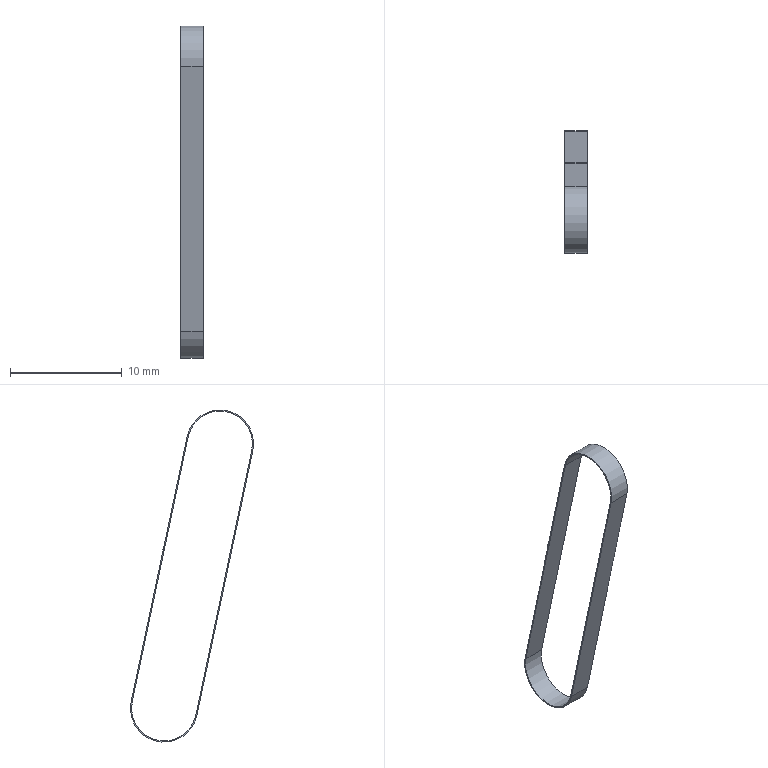Component | NX | BELT | 2 solids | 16 faces | box 2 x 11 x 29.68 mm | volume 13 mm3 | plane 12 | cylinder 4 | commonest cylinder face diameters 6 x2 5.8 x2
STEP:
#1=CARTESIAN_POINT('',(0.,0.,0.));
#2=DIRECTION('',(0.,0.,1.));
#3=DIRECTION('',(1.,0.,0.));
#4=AXIS2_PLACEMENT_3D('',#1,#2,#3);
#5=CARTESIAN_POINT('',(-47.1,-0.6394,30.62));
#6=VERTEX_POINT('',#5);
#7=CARTESIAN_POINT('',(-47.1,4.361,6.942));
#8=VERTEX_POINT('',#7);
#9=CARTESIAN_POINT('',(-47.1,4.361,6.942));
#10=DIRECTION('',(0.,0.2066,-0.9784));
#11=VECTOR('',#10,1.);
#12=LINE('',#9,#11);
#13=CARTESIAN_POINT('',(-47.1,4.263,6.921));
#14=DIRECTION('',(1.,0.,0.));
#15=DIRECTION('',(0.,-0.2066,0.9784));
#16=AXIS2_PLACEMENT_3D('',#13,#14,#15);
#17=PLANE('',#16);
#18=CARTESIAN_POINT('',(-0.,-0.1));
#19=DIRECTION('',(-1.,0.));
#20=VECTOR('',#19,1.);
#21=LINE('',#18,#20);
#22=(GEOMETRIC_REPRESENTATION_CONTEXT(2)PARAMETRIC_REPRESENTATION_CONTEXT()REPRESENTATION_CONTEXT('',''));
#23=DEFINITIONAL_REPRESENTATION('',(#21),#22);
#24=PCURVE('',#17,#23);
#25=CARTESIAN_POINT('',(-45.1,4.361,6.942));
#26=DIRECTION('',(0.,-0.9784,-0.2066));
#27=DIRECTION('',(1.,0.,0.));
#28=AXIS2_PLACEMENT_3D('',#25,#26,#27);
#29=PLANE('',#28);
#30=CARTESIAN_POINT('',(-2.,0.));
#31=DIRECTION('',(0.,-1.));
#32=VECTOR('',#31,1.);
#33=LINE('',#30,#32);
#34=(GEOMETRIC_REPRESENTATION_CONTEXT(2)PARAMETRIC_REPRESENTATION_CONTEXT()REPRESENTATION_CONTEXT('',''));
#35=DEFINITIONAL_REPRESENTATION('',(#33),#34);
#36=PCURVE('',#29,#35);
#37=SURFACE_CURVE('',#12,(#24,#36),.PCURVE_S1.);
#38=EDGE_CURVE('',#6,#8,#37,.T.);
#39=ORIENTED_EDGE('',*,*,#38,.T.);
#40=CARTESIAN_POINT('',(-47.1,-1.51,5.702));
#41=VERTEX_POINT('',#40);
#42=CARTESIAN_POINT('',(-47.1,1.425,6.322));
#43=DIRECTION('',(-1.,0.,0.));
#44=DIRECTION('',(0.,-0.9784,-0.2066));
#45=AXIS2_PLACEMENT_3D('',#42,#43,#44);
#46=CIRCLE('',#45,3.);
#47=CARTESIAN_POINT('',(-0.,5.9));
#48=CARTESIAN_POINT('',(5.196,5.9));
#49=CARTESIAN_POINT('',(2.598,1.4));
#50=CARTESIAN_POINT('',(-0.,-3.1));
#51=CARTESIAN_POINT('',(-2.598,1.4));
#52=CARTESIAN_POINT('',(-5.196,5.9));
#53=CARTESIAN_POINT('',(-0.,5.9));
#54=(BOUNDED_CURVE()B_SPLINE_CURVE(2,(#47,#48,#49,#50,#51,#52,#53),.UNSPECIFIED.,.T.,.F.)B_SPLINE_CURVE_WITH_KNOTS((1,2,2,2,2,1),(-2.094,0.,2.094,4.189,6.283,8.378),.UNSPECIFIED.)CURVE()GEOMETRIC_REPRESENTATION_ITEM()RATIONAL_B_SPLINE_CURVE((1.,0.5,1.,0.5,1.,0.5,1.))REPRESENTATION_ITEM(''));
#55=(GEOMETRIC_REPRESENTATION_CONTEXT(2)PARAMETRIC_REPRESENTATION_CONTEXT()REPRESENTATION_CONTEXT('',''));
#56=DEFINITIONAL_REPRESENTATION('',(#54),#55);
#57=PCURVE('',#17,#56);
#58=CARTESIAN_POINT('',(-45.1,1.425,6.322));
#59=DIRECTION('',(-1.,0.,0.));
#60=DIRECTION('',(0.,-0.9784,-0.2066));
#61=AXIS2_PLACEMENT_3D('',#58,#59,#60);
#62=CYLINDRICAL_SURFACE('',#61,3.);
#63=CARTESIAN_POINT('',(0.,2.));
#64=DIRECTION('',(1.,0.));
#65=VECTOR('',#64,1.);
#66=LINE('',#63,#65);
#67=(GEOMETRIC_REPRESENTATION_CONTEXT(2)PARAMETRIC_REPRESENTATION_CONTEXT()REPRESENTATION_CONTEXT('',''));
#68=DEFINITIONAL_REPRESENTATION('',(#66),#67);
#69=PCURVE('',#62,#68);
#70=SURFACE_CURVE('',#46,(#57,#69),.PCURVE_S1.);
#71=EDGE_CURVE('',#8,#41,#70,.T.);
#72=ORIENTED_EDGE('',*,*,#71,.T.);
#73=CARTESIAN_POINT('',(-47.1,-6.51,29.38));
#74=VERTEX_POINT('',#73);
#75=CARTESIAN_POINT('',(-47.1,-6.51,29.38));
#76=DIRECTION('',(0.,-0.2066,0.9784));
#77=VECTOR('',#76,1.);
#78=LINE('',#75,#77);
#79=CARTESIAN_POINT('',(24.2,5.9));
#80=DIRECTION('',(1.,0.));
#81=VECTOR('',#80,1.);
#82=LINE('',#79,#81);
#83=(GEOMETRIC_REPRESENTATION_CONTEXT(2)PARAMETRIC_REPRESENTATION_CONTEXT()REPRESENTATION_CONTEXT('',''));
#84=DEFINITIONAL_REPRESENTATION('',(#82),#83);
#85=PCURVE('',#17,#84);
#86=CARTESIAN_POINT('',(-45.1,-6.51,29.38));
#87=DIRECTION('',(0.,0.9784,0.2066));
#88=DIRECTION('',(-1.,0.,0.));
#89=AXIS2_PLACEMENT_3D('',#86,#87,#88);
#90=PLANE('',#89);
#91=CARTESIAN_POINT('',(2.,0.));
#92=DIRECTION('',(0.,1.));
#93=VECTOR('',#92,1.);
#94=LINE('',#91,#93);
#95=(GEOMETRIC_REPRESENTATION_CONTEXT(2)PARAMETRIC_REPRESENTATION_CONTEXT()REPRESENTATION_CONTEXT('',''));
#96=DEFINITIONAL_REPRESENTATION('',(#94),#95);
#97=PCURVE('',#90,#96);
#98=SURFACE_CURVE('',#78,(#85,#97),.PCURVE_S1.);
#99=EDGE_CURVE('',#41,#74,#98,.T.);
#100=ORIENTED_EDGE('',*,*,#99,.T.);
#101=CARTESIAN_POINT('',(-47.1,-3.575,30.));
#102=DIRECTION('',(-1.,0.,0.));
#103=DIRECTION('',(0.,-0.9784,-0.2066));
#104=AXIS2_PLACEMENT_3D('',#101,#102,#103);
#105=CIRCLE('',#104,3.);
#106=CARTESIAN_POINT('',(24.2,5.9));
#107=CARTESIAN_POINT('',(29.396,5.9));
#108=CARTESIAN_POINT('',(26.798,1.4));
#109=CARTESIAN_POINT('',(24.2,-3.1));
#110=CARTESIAN_POINT('',(21.602,1.4));
#111=CARTESIAN_POINT('',(19.004,5.9));
#112=CARTESIAN_POINT('',(24.2,5.9));
#113=(BOUNDED_CURVE()B_SPLINE_CURVE(2,(#106,#107,#108,#109,#110,#111,#112),.UNSPECIFIED.,.T.,.F.)B_SPLINE_CURVE_WITH_KNOTS((1,2,2,2,2,1),(-2.094,0.,2.094,4.189,6.283,8.378),.UNSPECIFIED.)CURVE()GEOMETRIC_REPRESENTATION_ITEM()RATIONAL_B_SPLINE_CURVE((1.,0.5,1.,0.5,1.,0.5,1.))REPRESENTATION_ITEM(''));
#114=(GEOMETRIC_REPRESENTATION_CONTEXT(2)PARAMETRIC_REPRESENTATION_CONTEXT()REPRESENTATION_CONTEXT('',''));
#115=DEFINITIONAL_REPRESENTATION('',(#113),#114);
#116=PCURVE('',#17,#115);
#117=CARTESIAN_POINT('',(-45.1,-3.575,30.));
#118=DIRECTION('',(-1.,0.,0.));
#119=DIRECTION('',(0.,-0.9784,-0.2066));
#120=AXIS2_PLACEMENT_3D('',#117,#118,#119);
#121=CYLINDRICAL_SURFACE('',#120,3.);
#122=CARTESIAN_POINT('',(0.,2.));
#123=DIRECTION('',(1.,0.));
#124=VECTOR('',#123,1.);
#125=LINE('',#122,#124);
#126=(GEOMETRIC_REPRESENTATION_CONTEXT(2)PARAMETRIC_REPRESENTATION_CONTEXT()REPRESENTATION_CONTEXT('',''));
#127=DEFINITIONAL_REPRESENTATION('',(#125),#126);
#128=PCURVE('',#121,#127);
#129=SURFACE_CURVE('',#105,(#116,#128),.PCURVE_S1.);
#130=EDGE_CURVE('',#74,#6,#129,.T.);
#131=ORIENTED_EDGE('',*,*,#130,.T.);
#132=EDGE_LOOP('',(#39,#72,#100,#131));
#133=FACE_BOUND('',#132,.T.);
#134=CARTESIAN_POINT('',(-47.1,4.263,6.921));
#135=VERTEX_POINT('',#134);
#136=CARTESIAN_POINT('',(-47.1,-0.7372,30.599));
#137=VERTEX_POINT('',#136);
#138=CARTESIAN_POINT('',(-47.1,4.263,6.921));
#139=DIRECTION('',(0.,-0.2066,0.9784));
#140=VECTOR('',#139,1.);
#141=LINE('',#138,#140);
#142=CARTESIAN_POINT('',(0.,0.));
#143=DIRECTION('',(1.,0.));
#144=VECTOR('',#143,1.);
#145=LINE('',#142,#144);
#146=(GEOMETRIC_REPRESENTATION_CONTEXT(2)PARAMETRIC_REPRESENTATION_CONTEXT()REPRESENTATION_CONTEXT('',''));
#147=DEFINITIONAL_REPRESENTATION('',(#145),#146);
#148=PCURVE('',#17,#147);
#149=CARTESIAN_POINT('',(-45.1,4.263,6.921));
#150=DIRECTION('',(0.,-0.9784,-0.2066));
#151=DIRECTION('',(1.,0.,0.));
#152=AXIS2_PLACEMENT_3D('',#149,#150,#151);
#153=PLANE('',#152);
#154=CARTESIAN_POINT('',(-2.,0.));
#155=DIRECTION('',(0.,1.));
#156=VECTOR('',#155,1.);
#157=LINE('',#154,#156);
#158=(GEOMETRIC_REPRESENTATION_CONTEXT(2)PARAMETRIC_REPRESENTATION_CONTEXT()REPRESENTATION_CONTEXT('',''));
#159=DEFINITIONAL_REPRESENTATION('',(#157),#158);
#160=PCURVE('',#153,#159);
#161=SURFACE_CURVE('',#141,(#148,#160),.PCURVE_S1.);
#162=EDGE_CURVE('',#135,#137,#161,.T.);
#163=ORIENTED_EDGE('',*,*,#162,.T.);
#164=CARTESIAN_POINT('',(-47.1,-6.412,29.401));
#165=VERTEX_POINT('',#164);
#166=CARTESIAN_POINT('',(-47.1,-3.575,30.));
#167=DIRECTION('',(1.,0.,0.));
#168=DIRECTION('',(0.,0.2066,-0.9784));
#169=AXIS2_PLACEMENT_3D('',#166,#167,#168);
#170=CIRCLE('',#169,2.9);
#171=CARTESIAN_POINT('',(24.2,2.9));
#172=DIRECTION('',(-1.,0.));
#173=AXIS2_PLACEMENT_2D('',#171,#172);
#174=CIRCLE('',#173,2.9);
#175=(GEOMETRIC_REPRESENTATION_CONTEXT(2)PARAMETRIC_REPRESENTATION_CONTEXT()REPRESENTATION_CONTEXT('',''));
#176=DEFINITIONAL_REPRESENTATION('',(#174),#175);
#177=PCURVE('',#17,#176);
#178=CARTESIAN_POINT('',(-45.1,-3.575,30.));
#179=DIRECTION('',(-1.,0.,0.));
#180=DIRECTION('',(0.,-0.9784,-0.2066));
#181=AXIS2_PLACEMENT_3D('',#178,#179,#180);
#182=CYLINDRICAL_SURFACE('',#181,2.9);
#183=CARTESIAN_POINT('',(4.712,2.));
#184=DIRECTION('',(-1.,0.));
#185=VECTOR('',#184,1.);
#186=LINE('',#183,#185);
#187=(GEOMETRIC_REPRESENTATION_CONTEXT(2)PARAMETRIC_REPRESENTATION_CONTEXT()REPRESENTATION_CONTEXT('',''));
#188=DEFINITIONAL_REPRESENTATION('',(#186),#187);
#189=PCURVE('',#182,#188);
#190=SURFACE_CURVE('',#170,(#177,#189),.PCURVE_S1.);
#191=EDGE_CURVE('',#137,#165,#190,.T.);
#192=ORIENTED_EDGE('',*,*,#191,.T.);
#193=CARTESIAN_POINT('',(-47.1,-1.412,5.723));
#194=VERTEX_POINT('',#193);
#195=CARTESIAN_POINT('',(-47.1,-6.412,29.401));
#196=DIRECTION('',(0.,0.2066,-0.9784));
#197=VECTOR('',#196,1.);
#198=LINE('',#195,#197);
#199=CARTESIAN_POINT('',(24.2,5.8));
#200=DIRECTION('',(-1.,0.));
#201=VECTOR('',#200,1.);
#202=LINE('',#199,#201);
#203=(GEOMETRIC_REPRESENTATION_CONTEXT(2)PARAMETRIC_REPRESENTATION_CONTEXT()REPRESENTATION_CONTEXT('',''));
#204=DEFINITIONAL_REPRESENTATION('',(#202),#203);
#205=PCURVE('',#17,#204);
#206=CARTESIAN_POINT('',(-45.1,-6.412,29.401));
#207=DIRECTION('',(0.,0.9784,0.2066));
#208=DIRECTION('',(-1.,0.,0.));
#209=AXIS2_PLACEMENT_3D('',#206,#207,#208);
#210=PLANE('',#209);
#211=CARTESIAN_POINT('',(2.,0.));
#212=DIRECTION('',(0.,-1.));
#213=VECTOR('',#212,1.);
#214=LINE('',#211,#213);
#215=(GEOMETRIC_REPRESENTATION_CONTEXT(2)PARAMETRIC_REPRESENTATION_CONTEXT()REPRESENTATION_CONTEXT('',''));
#216=DEFINITIONAL_REPRESENTATION('',(#214),#215);
#217=PCURVE('',#210,#216);
#218=SURFACE_CURVE('',#198,(#205,#217),.PCURVE_S1.);
#219=EDGE_CURVE('',#165,#194,#218,.T.);
#220=ORIENTED_EDGE('',*,*,#219,.T.);
#221=CARTESIAN_POINT('',(-47.1,1.425,6.322));
#222=DIRECTION('',(1.,0.,0.));
#223=DIRECTION('',(0.,-0.2066,0.9784));
#224=AXIS2_PLACEMENT_3D('',#221,#222,#223);
#225=CIRCLE('',#224,2.9);
#226=CARTESIAN_POINT('',(-0.,2.9));
#227=DIRECTION('',(1.,0.));
#228=AXIS2_PLACEMENT_2D('',#226,#227);
#229=CIRCLE('',#228,2.9);
#230=(GEOMETRIC_REPRESENTATION_CONTEXT(2)PARAMETRIC_REPRESENTATION_CONTEXT()REPRESENTATION_CONTEXT('',''));
#231=DEFINITIONAL_REPRESENTATION('',(#229),#230);
#232=PCURVE('',#17,#231);
#233=CARTESIAN_POINT('',(-45.1,1.425,6.322));
#234=DIRECTION('',(-1.,0.,0.));
#235=DIRECTION('',(0.,-0.9784,-0.2066));
#236=AXIS2_PLACEMENT_3D('',#233,#234,#235);
#237=CYLINDRICAL_SURFACE('',#236,2.9);
#238=CARTESIAN_POINT('',(7.854,2.));
#239=DIRECTION('',(-1.,0.));
#240=VECTOR('',#239,1.);
#241=LINE('',#238,#240);
#242=(GEOMETRIC_REPRESENTATION_CONTEXT(2)PARAMETRIC_REPRESENTATION_CONTEXT()REPRESENTATION_CONTEXT('',''));
#243=DEFINITIONAL_REPRESENTATION('',(#241),#242);
#244=PCURVE('',#237,#243);
#245=SURFACE_CURVE('',#225,(#232,#244),.PCURVE_S1.);
#246=EDGE_CURVE('',#194,#135,#245,.T.);
#247=ORIENTED_EDGE('',*,*,#246,.T.);
#248=EDGE_LOOP('',(#163,#192,#220,#247));
#249=FACE_BOUND('',#248,.T.);
#250=ADVANCED_FACE('',(#133,#249),#17,.F.);
#251=CARTESIAN_POINT('',(-45.1,-1.51,5.702));
#252=VERTEX_POINT('',#251);
#253=CARTESIAN_POINT('',(-45.1,-6.51,29.38));
#254=VERTEX_POINT('',#253);
#255=CARTESIAN_POINT('',(-45.1,-6.51,29.38));
#256=DIRECTION('',(0.,-0.2066,0.9784));
#257=VECTOR('',#256,1.);
#258=LINE('',#255,#257);
#259=CARTESIAN_POINT('',(-45.1,-6.412,29.401));
#260=DIRECTION('',(1.,0.,0.));
#261=DIRECTION('',(0.,0.2066,-0.9784));
#262=AXIS2_PLACEMENT_3D('',#259,#260,#261);
#263=PLANE('',#262);
#264=CARTESIAN_POINT('',(0.,-0.1));
#265=DIRECTION('',(-1.,0.));
#266=VECTOR('',#265,1.);
#267=LINE('',#264,#266);
#268=(GEOMETRIC_REPRESENTATION_CONTEXT(2)PARAMETRIC_REPRESENTATION_CONTEXT()REPRESENTATION_CONTEXT('',''));
#269=DEFINITIONAL_REPRESENTATION('',(#267),#268);
#270=PCURVE('',#263,#269);
#271=CARTESIAN_POINT('',(0.,0.));
#272=DIRECTION('',(0.,1.));
#273=VECTOR('',#272,1.);
#274=LINE('',#271,#273);
#275=(GEOMETRIC_REPRESENTATION_CONTEXT(2)PARAMETRIC_REPRESENTATION_CONTEXT()REPRESENTATION_CONTEXT('',''));
#276=DEFINITIONAL_REPRESENTATION('',(#274),#275);
#277=PCURVE('',#90,#276);
#278=SURFACE_CURVE('',#258,(#270,#277),.PCURVE_S1.);
#279=EDGE_CURVE('',#252,#254,#278,.T.);
#280=ORIENTED_EDGE('',*,*,#279,.F.);
#281=CARTESIAN_POINT('',(-45.1,4.361,6.942));
#282=VERTEX_POINT('',#281);
#283=CARTESIAN_POINT('',(-45.1,1.425,6.322));
#284=DIRECTION('',(-1.,0.,0.));
#285=DIRECTION('',(0.,-0.9784,-0.2066));
#286=AXIS2_PLACEMENT_3D('',#283,#284,#285);
#287=CIRCLE('',#286,3.);
#288=CARTESIAN_POINT('',(24.2,-0.1));
#289=CARTESIAN_POINT('',(19.004,-0.1));
#290=CARTESIAN_POINT('',(21.602,4.4));
#291=CARTESIAN_POINT('',(24.2,8.9));
#292=CARTESIAN_POINT('',(26.798,4.4));
#293=CARTESIAN_POINT('',(29.396,-0.1));
#294=CARTESIAN_POINT('',(24.2,-0.1));
#295=(BOUNDED_CURVE()B_SPLINE_CURVE(2,(#288,#289,#290,#291,#292,#293,#294),.UNSPECIFIED.,.T.,.F.)B_SPLINE_CURVE_WITH_KNOTS((1,2,2,2,2,1),(-2.094,0.,2.094,4.189,6.283,8.378),.UNSPECIFIED.)CURVE()GEOMETRIC_REPRESENTATION_ITEM()RATIONAL_B_SPLINE_CURVE((1.,0.5,1.,0.5,1.,0.5,1.))REPRESENTATION_ITEM(''));
#296=(GEOMETRIC_REPRESENTATION_CONTEXT(2)PARAMETRIC_REPRESENTATION_CONTEXT()REPRESENTATION_CONTEXT('',''));
#297=DEFINITIONAL_REPRESENTATION('',(#295),#296);
#298=PCURVE('',#263,#297);
#299=CARTESIAN_POINT('',(0.,0.));
#300=DIRECTION('',(1.,0.));
#301=VECTOR('',#300,1.);
#302=LINE('',#299,#301);
#303=(GEOMETRIC_REPRESENTATION_CONTEXT(2)PARAMETRIC_REPRESENTATION_CONTEXT()REPRESENTATION_CONTEXT('',''));
#304=DEFINITIONAL_REPRESENTATION('',(#302),#303);
#305=PCURVE('',#62,#304);
#306=SURFACE_CURVE('',#287,(#298,#305),.PCURVE_S1.);
#307=EDGE_CURVE('',#282,#252,#306,.T.);
#308=ORIENTED_EDGE('',*,*,#307,.F.);
#309=CARTESIAN_POINT('',(-45.1,-0.6394,30.62));
#310=VERTEX_POINT('',#309);
#311=CARTESIAN_POINT('',(-45.1,4.361,6.942));
#312=DIRECTION('',(0.,0.2066,-0.9784));
#313=VECTOR('',#312,1.);
#314=LINE('',#311,#313);
#315=CARTESIAN_POINT('',(24.2,5.9));
#316=DIRECTION('',(1.,0.));
#317=VECTOR('',#316,1.);
#318=LINE('',#315,#317);
#319=(GEOMETRIC_REPRESENTATION_CONTEXT(2)PARAMETRIC_REPRESENTATION_CONTEXT()REPRESENTATION_CONTEXT('',''));
#320=DEFINITIONAL_REPRESENTATION('',(#318),#319);
#321=PCURVE('',#263,#320);
#322=CARTESIAN_POINT('',(0.,0.));
#323=DIRECTION('',(0.,-1.));
#324=VECTOR('',#323,1.);
#325=LINE('',#322,#324);
#326=(GEOMETRIC_REPRESENTATION_CONTEXT(2)PARAMETRIC_REPRESENTATION_CONTEXT()REPRESENTATION_CONTEXT('',''));
#327=DEFINITIONAL_REPRESENTATION('',(#325),#326);
#328=PCURVE('',#29,#327);
#329=SURFACE_CURVE('',#314,(#321,#328),.PCURVE_S1.);
#330=EDGE_CURVE('',#310,#282,#329,.T.);
#331=ORIENTED_EDGE('',*,*,#330,.F.);
#332=CARTESIAN_POINT('',(-45.1,-3.575,30.));
#333=DIRECTION('',(-1.,0.,0.));
#334=DIRECTION('',(0.,-0.9784,-0.2066));
#335=AXIS2_PLACEMENT_3D('',#332,#333,#334);
#336=CIRCLE('',#335,3.);
#337=CARTESIAN_POINT('',(0.,-0.1));
#338=CARTESIAN_POINT('',(-5.196,-0.1));
#339=CARTESIAN_POINT('',(-2.598,4.4));
#340=CARTESIAN_POINT('',(0.,8.9));
#341=CARTESIAN_POINT('',(2.598,4.4));
#342=CARTESIAN_POINT('',(5.196,-0.1));
#343=CARTESIAN_POINT('',(0.,-0.1));
#344=(BOUNDED_CURVE()B_SPLINE_CURVE(2,(#337,#338,#339,#340,#341,#342,#343),.UNSPECIFIED.,.T.,.F.)B_SPLINE_CURVE_WITH_KNOTS((1,2,2,2,2,1),(-2.094,0.,2.094,4.189,6.283,8.378),.UNSPECIFIED.)CURVE()GEOMETRIC_REPRESENTATION_ITEM()RATIONAL_B_SPLINE_CURVE((1.,0.5,1.,0.5,1.,0.5,1.))REPRESENTATION_ITEM(''));
#345=(GEOMETRIC_REPRESENTATION_CONTEXT(2)PARAMETRIC_REPRESENTATION_CONTEXT()REPRESENTATION_CONTEXT('',''));
#346=DEFINITIONAL_REPRESENTATION('',(#344),#345);
#347=PCURVE('',#263,#346);
#348=CARTESIAN_POINT('',(0.,0.));
#349=DIRECTION('',(1.,0.));
#350=VECTOR('',#349,1.);
#351=LINE('',#348,#350);
#352=(GEOMETRIC_REPRESENTATION_CONTEXT(2)PARAMETRIC_REPRESENTATION_CONTEXT()REPRESENTATION_CONTEXT('',''));
#353=DEFINITIONAL_REPRESENTATION('',(#351),#352);
#354=PCURVE('',#121,#353);
#355=SURFACE_CURVE('',#336,(#347,#354),.PCURVE_S1.);
#356=EDGE_CURVE('',#254,#310,#355,.T.);
#357=ORIENTED_EDGE('',*,*,#356,.F.);
#358=EDGE_LOOP('',(#280,#308,#331,#357));
#359=FACE_BOUND('',#358,.T.);
#360=CARTESIAN_POINT('',(-45.1,-6.412,29.401));
#361=VERTEX_POINT('',#360);
#362=CARTESIAN_POINT('',(-45.1,-1.412,5.723));
#363=VERTEX_POINT('',#362);
#364=CARTESIAN_POINT('',(-45.1,-6.412,29.401));
#365=DIRECTION('',(0.,0.2066,-0.9784));
#366=VECTOR('',#365,1.);
#367=LINE('',#364,#366);
#368=CARTESIAN_POINT('',(0.,0.));
#369=DIRECTION('',(1.,0.));
#370=VECTOR('',#369,1.);
#371=LINE('',#368,#370);
#372=(GEOMETRIC_REPRESENTATION_CONTEXT(2)PARAMETRIC_REPRESENTATION_CONTEXT()REPRESENTATION_CONTEXT('',''));
#373=DEFINITIONAL_REPRESENTATION('',(#371),#372);
#374=PCURVE('',#263,#373);
#375=CARTESIAN_POINT('',(0.,0.));
#376=DIRECTION('',(0.,-1.));
#377=VECTOR('',#376,1.);
#378=LINE('',#375,#377);
#379=(GEOMETRIC_REPRESENTATION_CONTEXT(2)PARAMETRIC_REPRESENTATION_CONTEXT()REPRESENTATION_CONTEXT('',''));
#380=DEFINITIONAL_REPRESENTATION('',(#378),#379);
#381=PCURVE('',#210,#380);
#382=SURFACE_CURVE('',#367,(#374,#381),.PCURVE_S1.);
#383=EDGE_CURVE('',#361,#363,#382,.T.);
#384=ORIENTED_EDGE('',*,*,#383,.F.);
#385=CARTESIAN_POINT('',(-45.1,-0.7372,30.599));
#386=VERTEX_POINT('',#385);
#387=CARTESIAN_POINT('',(-45.1,-3.575,30.));
#388=DIRECTION('',(1.,0.,0.));
#389=DIRECTION('',(0.,0.2066,-0.9784));
#390=AXIS2_PLACEMENT_3D('',#387,#388,#389);
#391=CIRCLE('',#390,2.9);
#392=CARTESIAN_POINT('',(0.,2.9));
#393=DIRECTION('',(1.,-0.));
#394=AXIS2_PLACEMENT_2D('',#392,#393);
#395=CIRCLE('',#394,2.9);
#396=(GEOMETRIC_REPRESENTATION_CONTEXT(2)PARAMETRIC_REPRESENTATION_CONTEXT()REPRESENTATION_CONTEXT('',''));
#397=DEFINITIONAL_REPRESENTATION('',(#395),#396);
#398=PCURVE('',#263,#397);
#399=CARTESIAN_POINT('',(4.712,0.));
#400=DIRECTION('',(-1.,0.));
#401=VECTOR('',#400,1.);
#402=LINE('',#399,#401);
#403=(GEOMETRIC_REPRESENTATION_CONTEXT(2)PARAMETRIC_REPRESENTATION_CONTEXT()REPRESENTATION_CONTEXT('',''));
#404=DEFINITIONAL_REPRESENTATION('',(#402),#403);
#405=PCURVE('',#182,#404);
#406=SURFACE_CURVE('',#391,(#398,#405),.PCURVE_S1.);
#407=EDGE_CURVE('',#386,#361,#406,.T.);
#408=ORIENTED_EDGE('',*,*,#407,.F.);
#409=CARTESIAN_POINT('',(-45.1,4.263,6.921));
#410=VERTEX_POINT('',#409);
#411=CARTESIAN_POINT('',(-45.1,4.263,6.921));
#412=DIRECTION('',(0.,-0.2066,0.9784));
#413=VECTOR('',#412,1.);
#414=LINE('',#411,#413);
#415=CARTESIAN_POINT('',(24.2,5.8));
#416=DIRECTION('',(-1.,0.));
#417=VECTOR('',#416,1.);
#418=LINE('',#415,#417);
#419=(GEOMETRIC_REPRESENTATION_CONTEXT(2)PARAMETRIC_REPRESENTATION_CONTEXT()REPRESENTATION_CONTEXT('',''));
#420=DEFINITIONAL_REPRESENTATION('',(#418),#419);
#421=PCURVE('',#263,#420);
#422=CARTESIAN_POINT('',(0.,0.));
#423=DIRECTION('',(0.,1.));
#424=VECTOR('',#423,1.);
#425=LINE('',#422,#424);
#426=(GEOMETRIC_REPRESENTATION_CONTEXT(2)PARAMETRIC_REPRESENTATION_CONTEXT()REPRESENTATION_CONTEXT('',''));
#427=DEFINITIONAL_REPRESENTATION('',(#425),#426);
#428=PCURVE('',#153,#427);
#429=SURFACE_CURVE('',#414,(#421,#428),.PCURVE_S1.);
#430=EDGE_CURVE('',#410,#386,#429,.T.);
#431=ORIENTED_EDGE('',*,*,#430,.F.);
#432=CARTESIAN_POINT('',(-45.1,1.425,6.322));
#433=DIRECTION('',(1.,0.,0.));
#434=DIRECTION('',(0.,-0.2066,0.9784));
#435=AXIS2_PLACEMENT_3D('',#432,#433,#434);
#436=CIRCLE('',#435,2.9);
#437=CARTESIAN_POINT('',(24.2,2.9));
#438=DIRECTION('',(-1.,0.));
#439=AXIS2_PLACEMENT_2D('',#437,#438);
#440=CIRCLE('',#439,2.9);
#441=(GEOMETRIC_REPRESENTATION_CONTEXT(2)PARAMETRIC_REPRESENTATION_CONTEXT()REPRESENTATION_CONTEXT('',''));
#442=DEFINITIONAL_REPRESENTATION('',(#440),#441);
#443=PCURVE('',#263,#442);
#444=CARTESIAN_POINT('',(7.854,0.));
#445=DIRECTION('',(-1.,0.));
#446=VECTOR('',#445,1.);
#447=LINE('',#444,#446);
#448=(GEOMETRIC_REPRESENTATION_CONTEXT(2)PARAMETRIC_REPRESENTATION_CONTEXT()REPRESENTATION_CONTEXT('',''));
#449=DEFINITIONAL_REPRESENTATION('',(#447),#448);
#450=PCURVE('',#237,#449);
#451=SURFACE_CURVE('',#436,(#443,#450),.PCURVE_S1.);
#452=EDGE_CURVE('',#363,#410,#451,.T.);
#453=ORIENTED_EDGE('',*,*,#452,.F.);
#454=EDGE_LOOP('',(#384,#408,#431,#453));
#455=FACE_BOUND('',#454,.T.);
#456=ADVANCED_FACE('',(#359,#455),#263,.T.);
#457=ORIENTED_EDGE('',*,*,#71,.F.);
#458=CARTESIAN_POINT('',(-45.1,4.361,6.942));
#459=DIRECTION('',(-1.,0.,0.));
#460=VECTOR('',#459,1.);
#461=LINE('',#458,#460);
#462=CARTESIAN_POINT('',(3.142,0.));
#463=DIRECTION('',(0.,1.));
#464=VECTOR('',#463,1.);
#465=LINE('',#462,#464);
#466=(GEOMETRIC_REPRESENTATION_CONTEXT(2)PARAMETRIC_REPRESENTATION_CONTEXT()REPRESENTATION_CONTEXT('',''));
#467=DEFINITIONAL_REPRESENTATION('',(#465),#466);
#468=PCURVE('',#62,#467);
#469=CARTESIAN_POINT('',(0.,0.));
#470=DIRECTION('',(-1.,0.));
#471=VECTOR('',#470,1.);
#472=LINE('',#469,#471);
#473=(GEOMETRIC_REPRESENTATION_CONTEXT(2)PARAMETRIC_REPRESENTATION_CONTEXT()REPRESENTATION_CONTEXT('',''));
#474=DEFINITIONAL_REPRESENTATION('',(#472),#473);
#475=PCURVE('',#29,#474);
#476=SURFACE_CURVE('',#461,(#468,#475),.PCURVE_S1.);
#477=EDGE_CURVE('',#282,#8,#476,.T.);
#478=ORIENTED_EDGE('',*,*,#477,.F.);
#479=ORIENTED_EDGE('',*,*,#307,.T.);
#480=CARTESIAN_POINT('',(-45.1,-1.51,5.702));
#481=DIRECTION('',(-1.,0.,0.));
#482=VECTOR('',#481,1.);
#483=LINE('',#480,#482);
#484=CARTESIAN_POINT('',(6.283,0.));
#485=DIRECTION('',(0.,1.));
#486=VECTOR('',#485,1.);
#487=LINE('',#484,#486);
#488=(GEOMETRIC_REPRESENTATION_CONTEXT(2)PARAMETRIC_REPRESENTATION_CONTEXT()REPRESENTATION_CONTEXT('',''));
#489=DEFINITIONAL_REPRESENTATION('',(#487),#488);
#490=PCURVE('',#62,#489);
#491=CARTESIAN_POINT('',(0.,-24.2));
#492=DIRECTION('',(1.,0.));
#493=VECTOR('',#492,1.);
#494=LINE('',#491,#493);
#495=(GEOMETRIC_REPRESENTATION_CONTEXT(2)PARAMETRIC_REPRESENTATION_CONTEXT()REPRESENTATION_CONTEXT('',''));
#496=DEFINITIONAL_REPRESENTATION('',(#494),#495);
#497=PCURVE('',#90,#496);
#498=SURFACE_CURVE('',#483,(#490,#497),.PCURVE_S1.);
#499=EDGE_CURVE('',#252,#41,#498,.T.);
#500=ORIENTED_EDGE('',*,*,#499,.T.);
#501=EDGE_LOOP('',(#457,#478,#479,#500));
#502=FACE_BOUND('',#501,.T.);
#503=ADVANCED_FACE('',(#502),#62,.T.);
#504=ORIENTED_EDGE('',*,*,#38,.F.);
#505=CARTESIAN_POINT('',(-45.1,-0.6394,30.62));
#506=DIRECTION('',(-1.,0.,0.));
#507=VECTOR('',#506,1.);
#508=LINE('',#505,#507);
#509=CARTESIAN_POINT('',(0.,24.2));
#510=DIRECTION('',(-1.,0.));
#511=VECTOR('',#510,1.);
#512=LINE('',#509,#511);
#513=(GEOMETRIC_REPRESENTATION_CONTEXT(2)PARAMETRIC_REPRESENTATION_CONTEXT()REPRESENTATION_CONTEXT('',''));
#514=DEFINITIONAL_REPRESENTATION('',(#512),#513);
#515=PCURVE('',#29,#514);
#516=CARTESIAN_POINT('',(3.142,0.));
#517=DIRECTION('',(0.,1.));
#518=VECTOR('',#517,1.);
#519=LINE('',#516,#518);
#520=(GEOMETRIC_REPRESENTATION_CONTEXT(2)PARAMETRIC_REPRESENTATION_CONTEXT()REPRESENTATION_CONTEXT('',''));
#521=DEFINITIONAL_REPRESENTATION('',(#519),#520);
#522=PCURVE('',#121,#521);
#523=SURFACE_CURVE('',#508,(#515,#522),.PCURVE_S1.);
#524=EDGE_CURVE('',#310,#6,#523,.T.);
#525=ORIENTED_EDGE('',*,*,#524,.F.);
#526=ORIENTED_EDGE('',*,*,#330,.T.);
#527=ORIENTED_EDGE('',*,*,#477,.T.);
#528=EDGE_LOOP('',(#504,#525,#526,#527));
#529=FACE_BOUND('',#528,.T.);
#530=ADVANCED_FACE('',(#529),#29,.F.);
#531=ORIENTED_EDGE('',*,*,#130,.F.);
#532=CARTESIAN_POINT('',(-45.1,-6.51,29.38));
#533=DIRECTION('',(-1.,0.,0.));
#534=VECTOR('',#533,1.);
#535=LINE('',#532,#534);
#536=CARTESIAN_POINT('',(0.,0.));
#537=DIRECTION('',(0.,1.));
#538=VECTOR('',#537,1.);
#539=LINE('',#536,#538);
#540=(GEOMETRIC_REPRESENTATION_CONTEXT(2)PARAMETRIC_REPRESENTATION_CONTEXT()REPRESENTATION_CONTEXT('',''));
#541=DEFINITIONAL_REPRESENTATION('',(#539),#540);
#542=PCURVE('',#121,#541);
#543=CARTESIAN_POINT('',(0.,0.));
#544=DIRECTION('',(1.,0.));
#545=VECTOR('',#544,1.);
#546=LINE('',#543,#545);
#547=(GEOMETRIC_REPRESENTATION_CONTEXT(2)PARAMETRIC_REPRESENTATION_CONTEXT()REPRESENTATION_CONTEXT('',''));
#548=DEFINITIONAL_REPRESENTATION('',(#546),#547);
#549=PCURVE('',#90,#548);
#550=SURFACE_CURVE('',#535,(#542,#549),.PCURVE_S1.);
#551=EDGE_CURVE('',#254,#74,#550,.T.);
#552=ORIENTED_EDGE('',*,*,#551,.F.);
#553=ORIENTED_EDGE('',*,*,#356,.T.);
#554=ORIENTED_EDGE('',*,*,#524,.T.);
#555=EDGE_LOOP('',(#531,#552,#553,#554));
#556=FACE_BOUND('',#555,.T.);
#557=ADVANCED_FACE('',(#556),#121,.T.);
#558=ORIENTED_EDGE('',*,*,#99,.F.);
#559=ORIENTED_EDGE('',*,*,#499,.F.);
#560=ORIENTED_EDGE('',*,*,#279,.T.);
#561=ORIENTED_EDGE('',*,*,#551,.T.);
#562=EDGE_LOOP('',(#558,#559,#560,#561));
#563=FACE_BOUND('',#562,.T.);
#564=ADVANCED_FACE('',(#563),#90,.F.);
#565=CARTESIAN_POINT('',(-45.1,4.263,6.921));
#566=DIRECTION('',(-1.,0.,0.));
#567=VECTOR('',#566,1.);
#568=LINE('',#565,#567);
#569=CARTESIAN_POINT('',(3.142,0.));
#570=DIRECTION('',(0.,1.));
#571=VECTOR('',#570,1.);
#572=LINE('',#569,#571);
#573=(GEOMETRIC_REPRESENTATION_CONTEXT(2)PARAMETRIC_REPRESENTATION_CONTEXT()REPRESENTATION_CONTEXT('',''));
#574=DEFINITIONAL_REPRESENTATION('',(#572),#573);
#575=PCURVE('',#237,#574);
#576=CARTESIAN_POINT('',(0.,0.));
#577=DIRECTION('',(-1.,0.));
#578=VECTOR('',#577,1.);
#579=LINE('',#576,#578);
#580=(GEOMETRIC_REPRESENTATION_CONTEXT(2)PARAMETRIC_REPRESENTATION_CONTEXT()REPRESENTATION_CONTEXT('',''));
#581=DEFINITIONAL_REPRESENTATION('',(#579),#580);
#582=PCURVE('',#153,#581);
#583=SURFACE_CURVE('',#568,(#575,#582),.PCURVE_S1.);
#584=EDGE_CURVE('',#410,#135,#583,.T.);
#585=ORIENTED_EDGE('',*,*,#584,.F.);
#586=ORIENTED_EDGE('',*,*,#452,.F.);
#587=CARTESIAN_POINT('',(-45.1,-1.412,5.723));
#588=DIRECTION('',(-1.,0.,0.));
#589=VECTOR('',#588,1.);
#590=LINE('',#587,#589);
#591=CARTESIAN_POINT('',(6.283,0.));
#592=DIRECTION('',(0.,1.));
#593=VECTOR('',#592,1.);
#594=LINE('',#591,#593);
#595=(GEOMETRIC_REPRESENTATION_CONTEXT(2)PARAMETRIC_REPRESENTATION_CONTEXT()REPRESENTATION_CONTEXT('',''));
#596=DEFINITIONAL_REPRESENTATION('',(#594),#595);
#597=PCURVE('',#237,#596);
#598=CARTESIAN_POINT('',(0.,-24.2));
#599=DIRECTION('',(1.,0.));
#600=VECTOR('',#599,1.);
#601=LINE('',#598,#600);
#602=(GEOMETRIC_REPRESENTATION_CONTEXT(2)PARAMETRIC_REPRESENTATION_CONTEXT()REPRESENTATION_CONTEXT('',''));
#603=DEFINITIONAL_REPRESENTATION('',(#601),#602);
#604=PCURVE('',#210,#603);
#605=SURFACE_CURVE('',#590,(#597,#604),.PCURVE_S1.);
#606=EDGE_CURVE('',#363,#194,#605,.T.);
#607=ORIENTED_EDGE('',*,*,#606,.T.);
#608=ORIENTED_EDGE('',*,*,#246,.T.);
#609=EDGE_LOOP('',(#585,#586,#607,#608));
#610=FACE_BOUND('',#609,.F.);
#611=ADVANCED_FACE('',(#610),#237,.F.);
#612=ORIENTED_EDGE('',*,*,#162,.F.);
#613=ORIENTED_EDGE('',*,*,#584,.F.);
#614=ORIENTED_EDGE('',*,*,#430,.T.);
#615=CARTESIAN_POINT('',(-45.1,-0.7372,30.599));
#616=DIRECTION('',(-1.,0.,0.));
#617=VECTOR('',#616,1.);
#618=LINE('',#615,#617);
#619=CARTESIAN_POINT('',(0.,24.2));
#620=DIRECTION('',(-1.,0.));
#621=VECTOR('',#620,1.);
#622=LINE('',#619,#621);
#623=(GEOMETRIC_REPRESENTATION_CONTEXT(2)PARAMETRIC_REPRESENTATION_CONTEXT()REPRESENTATION_CONTEXT('',''));
#624=DEFINITIONAL_REPRESENTATION('',(#622),#623);
#625=PCURVE('',#153,#624);
#626=CARTESIAN_POINT('',(3.142,0.));
#627=DIRECTION('',(0.,1.));
#628=VECTOR('',#627,1.);
#629=LINE('',#626,#628);
#630=(GEOMETRIC_REPRESENTATION_CONTEXT(2)PARAMETRIC_REPRESENTATION_CONTEXT()REPRESENTATION_CONTEXT('',''));
#631=DEFINITIONAL_REPRESENTATION('',(#629),#630);
#632=PCURVE('',#182,#631);
#633=SURFACE_CURVE('',#618,(#625,#632),.PCURVE_S1.);
#634=EDGE_CURVE('',#386,#137,#633,.T.);
#635=ORIENTED_EDGE('',*,*,#634,.T.);
#636=EDGE_LOOP('',(#612,#613,#614,#635));
#637=FACE_BOUND('',#636,.T.);
#638=ADVANCED_FACE('',(#637),#153,.T.);
#639=CARTESIAN_POINT('',(-45.1,-6.412,29.401));
#640=DIRECTION('',(-1.,0.,0.));
#641=VECTOR('',#640,1.);
#642=LINE('',#639,#641);
#643=CARTESIAN_POINT('',(0.,0.));
#644=DIRECTION('',(0.,1.));
#645=VECTOR('',#644,1.);
#646=LINE('',#643,#645);
#647=(GEOMETRIC_REPRESENTATION_CONTEXT(2)PARAMETRIC_REPRESENTATION_CONTEXT()REPRESENTATION_CONTEXT('',''));
#648=DEFINITIONAL_REPRESENTATION('',(#646),#647);
#649=PCURVE('',#182,#648);
#650=CARTESIAN_POINT('',(0.,0.));
#651=DIRECTION('',(1.,0.));
#652=VECTOR('',#651,1.);
#653=LINE('',#650,#652);
#654=(GEOMETRIC_REPRESENTATION_CONTEXT(2)PARAMETRIC_REPRESENTATION_CONTEXT()REPRESENTATION_CONTEXT('',''));
#655=DEFINITIONAL_REPRESENTATION('',(#653),#654);
#656=PCURVE('',#210,#655);
#657=SURFACE_CURVE('',#642,(#649,#656),.PCURVE_S1.);
#658=EDGE_CURVE('',#361,#165,#657,.T.);
#659=ORIENTED_EDGE('',*,*,#658,.F.);
#660=ORIENTED_EDGE('',*,*,#407,.F.);
#661=ORIENTED_EDGE('',*,*,#634,.T.);
#662=ORIENTED_EDGE('',*,*,#191,.T.);
#663=EDGE_LOOP('',(#659,#660,#661,#662));
#664=FACE_BOUND('',#663,.F.);
#665=ADVANCED_FACE('',(#664),#182,.F.);
#666=ORIENTED_EDGE('',*,*,#219,.F.);
#667=ORIENTED_EDGE('',*,*,#658,.F.);
#668=ORIENTED_EDGE('',*,*,#383,.T.);
#669=ORIENTED_EDGE('',*,*,#606,.T.);
#670=EDGE_LOOP('',(#666,#667,#668,#669));
#671=FACE_BOUND('',#670,.T.);
#672=ADVANCED_FACE('',(#671),#210,.T.);
#673=CLOSED_SHELL('',(#250,#456,#503,#530,#557,#564,#611,#638,#665,#672));
#674=MANIFOLD_SOLID_BREP('',#673);
#675=(LENGTH_UNIT()NAMED_UNIT(*)SI_UNIT(.MILLI.,.METRE.));
#676=UNCERTAINTY_MEASURE_WITH_UNIT(LENGTH_MEASURE(0.0000001),#675,'','');
#677=(NAMED_UNIT(*)PLANE_ANGLE_UNIT()SI_UNIT($,.RADIAN.));
#678=(NAMED_UNIT(*)SI_UNIT($,.STERADIAN.)SOLID_ANGLE_UNIT());
#679=(GEOMETRIC_REPRESENTATION_CONTEXT(3)GLOBAL_UNCERTAINTY_ASSIGNED_CONTEXT((#676))GLOBAL_UNIT_ASSIGNED_CONTEXT((#675,#677,#678))REPRESENTATION_CONTEXT('',''));
#680=ADVANCED_BREP_SHAPE_REPRESENTATION('',(#4,#674),#679);
#681=CARTESIAN_POINT('',(0.,0.,0.));
#682=DIRECTION('',(0.,0.,1.));
#683=DIRECTION('',(1.,0.,0.));
#684=AXIS2_PLACEMENT_3D('',#681,#682,#683);
#685=CARTESIAN_POINT('',(0.,0.,0.));
#686=DIRECTION('',(0.,0.,1.));
#687=DIRECTION('',(1.,0.,0.));
#688=AXIS2_PLACEMENT_3D('',#685,#686,#687);
#689=(LENGTH_UNIT()NAMED_UNIT(*)SI_UNIT(.MILLI.,.METRE.));
#690=UNCERTAINTY_MEASURE_WITH_UNIT(LENGTH_MEASURE(0.0000001),#689,'','');
#691=(NAMED_UNIT(*)PLANE_ANGLE_UNIT()SI_UNIT($,.RADIAN.));
#692=(NAMED_UNIT(*)SI_UNIT($,.STERADIAN.)SOLID_ANGLE_UNIT());
#693=(GEOMETRIC_REPRESENTATION_CONTEXT(3)GLOBAL_UNCERTAINTY_ASSIGNED_CONTEXT((#690))GLOBAL_UNIT_ASSIGNED_CONTEXT((#689,#691,#692))REPRESENTATION_CONTEXT('',''));
#694=SHAPE_REPRESENTATION('',(#4,#684,#688),#693);
#695=ITEM_DEFINED_TRANSFORMATION('','',#4,#684);
#696=(REPRESENTATION_RELATIONSHIP('','',#680,#694)REPRESENTATION_RELATIONSHIP_WITH_TRANSFORMATION(#695)SHAPE_REPRESENTATION_RELATIONSHIP());
#697=CARTESIAN_POINT('',(-47.1,1.434,20.802));
#698=VERTEX_POINT('',#697);
#699=CARTESIAN_POINT('',(-45.1,1.434,20.802));
#700=VERTEX_POINT('',#699);
#701=CARTESIAN_POINT('',(-47.1,1.434,20.802));
#702=DIRECTION('',(1.,0.,0.));
#703=VECTOR('',#702,1.);
#704=LINE('',#701,#703);
#705=CARTESIAN_POINT('',(-47.1,1.483,20.812));
#706=DIRECTION('',(0.,0.2066,-0.9784));
#707=DIRECTION('',(0.,0.9784,0.2066));
#708=AXIS2_PLACEMENT_3D('',#705,#706,#707);
#709=PLANE('',#708);
#710=CARTESIAN_POINT('',(-0.05,0.));
#711=DIRECTION('',(0.,1.));
#712=VECTOR('',#711,1.);
#713=LINE('',#710,#712);
#714=(GEOMETRIC_REPRESENTATION_CONTEXT(2)PARAMETRIC_REPRESENTATION_CONTEXT()REPRESENTATION_CONTEXT('',''));
#715=DEFINITIONAL_REPRESENTATION('',(#713),#714);
#716=PCURVE('',#709,#715);
#717=CARTESIAN_POINT('',(-46.1,1.861,18.781));
#718=DIRECTION('',(0.,0.9784,0.2066));
#719=DIRECTION('',(0.,-0.2066,0.9784));
#720=AXIS2_PLACEMENT_3D('',#717,#718,#719);
#721=PLANE('',#720);
#722=CARTESIAN_POINT('',(2.065,-1.));
#723=DIRECTION('',(0.,1.));
#724=VECTOR('',#723,1.);
#725=LINE('',#722,#724);
#726=(GEOMETRIC_REPRESENTATION_CONTEXT(2)PARAMETRIC_REPRESENTATION_CONTEXT()REPRESENTATION_CONTEXT('',''));
#727=DEFINITIONAL_REPRESENTATION('',(#725),#726);
#728=PCURVE('',#721,#727);
#729=SURFACE_CURVE('',#704,(#716,#728),.PCURVE_S1.);
#730=EDGE_CURVE('',#698,#700,#729,.T.);
#731=ORIENTED_EDGE('',*,*,#730,.T.);
#732=CARTESIAN_POINT('',(-45.1,1.483,20.812));
#733=VERTEX_POINT('',#732);
#734=CARTESIAN_POINT('',(-45.1,1.483,20.812));
#735=DIRECTION('',(0.,-0.9784,-0.2066));
#736=VECTOR('',#735,1.);
#737=LINE('',#734,#736);
#738=CARTESIAN_POINT('',(0.,2.));
#739=DIRECTION('',(-1.,0.));
#740=VECTOR('',#739,1.);
#741=LINE('',#738,#740);
#742=(GEOMETRIC_REPRESENTATION_CONTEXT(2)PARAMETRIC_REPRESENTATION_CONTEXT()REPRESENTATION_CONTEXT('',''));
#743=DEFINITIONAL_REPRESENTATION('',(#741),#742);
#744=PCURVE('',#709,#743);
#745=CARTESIAN_POINT('',(-45.1,1.483,20.812));
#746=DIRECTION('',(-1.,0.,0.));
#747=DIRECTION('',(0.,-0.9784,-0.2066));
#748=AXIS2_PLACEMENT_3D('',#745,#746,#747);
#749=PLANE('',#748);
#750=CARTESIAN_POINT('',(0.,0.));
#751=DIRECTION('',(1.,0.));
#752=VECTOR('',#751,1.);
#753=LINE('',#750,#752);
#754=(GEOMETRIC_REPRESENTATION_CONTEXT(2)PARAMETRIC_REPRESENTATION_CONTEXT()REPRESENTATION_CONTEXT('',''));
#755=DEFINITIONAL_REPRESENTATION('',(#753),#754);
#756=PCURVE('',#749,#755);
#757=SURFACE_CURVE('',#737,(#744,#756),.PCURVE_S1.);
#758=EDGE_CURVE('',#733,#700,#757,.T.);
#759=ORIENTED_EDGE('',*,*,#758,.F.);
#760=CARTESIAN_POINT('',(-47.1,1.483,20.812));
#761=VERTEX_POINT('',#760);
#762=CARTESIAN_POINT('',(-47.1,1.483,20.812));
#763=DIRECTION('',(1.,0.,0.));
#764=VECTOR('',#763,1.);
#765=LINE('',#762,#764);
#766=CARTESIAN_POINT('',(0.,0.));
#767=DIRECTION('',(0.,1.));
#768=VECTOR('',#767,1.);
#769=LINE('',#766,#768);
#770=(GEOMETRIC_REPRESENTATION_CONTEXT(2)PARAMETRIC_REPRESENTATION_CONTEXT()REPRESENTATION_CONTEXT('',''));
#771=DEFINITIONAL_REPRESENTATION('',(#769),#770);
#772=PCURVE('',#709,#771);
#773=CARTESIAN_POINT('',(-46.1,1.91,18.791));
#774=DIRECTION('',(0.,0.9784,0.2066));
#775=DIRECTION('',(0.,-0.2066,0.9784));
#776=AXIS2_PLACEMENT_3D('',#773,#774,#775);
#777=PLANE('',#776);
#778=CARTESIAN_POINT('',(2.065,-1.));
#779=DIRECTION('',(0.,1.));
#780=VECTOR('',#779,1.);
#781=LINE('',#778,#780);
#782=(GEOMETRIC_REPRESENTATION_CONTEXT(2)PARAMETRIC_REPRESENTATION_CONTEXT()REPRESENTATION_CONTEXT('',''));
#783=DEFINITIONAL_REPRESENTATION('',(#781),#782);
#784=PCURVE('',#777,#783);
#785=SURFACE_CURVE('',#765,(#772,#784),.PCURVE_S1.);
#786=EDGE_CURVE('',#761,#733,#785,.T.);
#787=ORIENTED_EDGE('',*,*,#786,.F.);
#788=CARTESIAN_POINT('',(-47.1,1.483,20.812));
#789=DIRECTION('',(0.,-0.9784,-0.2066));
#790=VECTOR('',#789,1.);
#791=LINE('',#788,#790);
#792=CARTESIAN_POINT('',(0.,0.));
#793=DIRECTION('',(-1.,0.));
#794=VECTOR('',#793,1.);
#795=LINE('',#792,#794);
#796=(GEOMETRIC_REPRESENTATION_CONTEXT(2)PARAMETRIC_REPRESENTATION_CONTEXT()REPRESENTATION_CONTEXT('',''));
#797=DEFINITIONAL_REPRESENTATION('',(#795),#796);
#798=PCURVE('',#709,#797);
#799=CARTESIAN_POINT('',(-47.1,1.538,20.55));
#800=DIRECTION('',(1.,0.,0.));
#801=DIRECTION('',(0.,0.9784,0.2066));
#802=AXIS2_PLACEMENT_3D('',#799,#800,#801);
#803=PLANE('',#802);
#804=CARTESIAN_POINT('',(0.,0.2677));
#805=DIRECTION('',(-1.,0.));
#806=VECTOR('',#805,1.);
#807=LINE('',#804,#806);
#808=(GEOMETRIC_REPRESENTATION_CONTEXT(2)PARAMETRIC_REPRESENTATION_CONTEXT()REPRESENTATION_CONTEXT('',''));
#809=DEFINITIONAL_REPRESENTATION('',(#807),#808);
#810=PCURVE('',#803,#809);
#811=SURFACE_CURVE('',#791,(#798,#810),.PCURVE_S1.);
#812=EDGE_CURVE('',#761,#698,#811,.T.);
#813=ORIENTED_EDGE('',*,*,#812,.T.);
#814=EDGE_LOOP('',(#731,#759,#787,#813));
#815=FACE_BOUND('',#814,.T.);
#816=ADVANCED_FACE('',(#815),#709,.F.);
#817=CARTESIAN_POINT('',(-45.1,1.489,20.54));
#818=VERTEX_POINT('',#817);
#819=CARTESIAN_POINT('',(-45.1,1.434,20.802));
#820=DIRECTION('',(0.,0.2066,-0.9784));
#821=VECTOR('',#820,1.);
#822=LINE('',#819,#821);
#823=CARTESIAN_POINT('',(0.05,-0.));
#824=DIRECTION('',(-0.,-1.));
#825=VECTOR('',#824,1.);
#826=LINE('',#823,#825);
#827=(GEOMETRIC_REPRESENTATION_CONTEXT(2)PARAMETRIC_REPRESENTATION_CONTEXT()REPRESENTATION_CONTEXT('',''));
#828=DEFINITIONAL_REPRESENTATION('',(#826),#827);
#829=PCURVE('',#749,#828);
#830=CARTESIAN_POINT('',(2.065,1.));
#831=DIRECTION('',(-1.,0.));
#832=VECTOR('',#831,1.);
#833=LINE('',#830,#832);
#834=(GEOMETRIC_REPRESENTATION_CONTEXT(2)PARAMETRIC_REPRESENTATION_CONTEXT()REPRESENTATION_CONTEXT('',''));
#835=DEFINITIONAL_REPRESENTATION('',(#833),#834);
#836=PCURVE('',#721,#835);
#837=SURFACE_CURVE('',#822,(#829,#836),.PCURVE_S1.);
#838=EDGE_CURVE('',#700,#818,#837,.T.);
#839=ORIENTED_EDGE('',*,*,#838,.T.);
#840=CARTESIAN_POINT('',(-45.1,1.538,20.55));
#841=VERTEX_POINT('',#840);
#842=CARTESIAN_POINT('',(-45.1,1.538,20.55));
#843=DIRECTION('',(0.,-0.9784,-0.2066));
#844=VECTOR('',#843,1.);
#845=LINE('',#842,#844);
#846=CARTESIAN_POINT('',(0.,-0.2677));
#847=DIRECTION('',(1.,0.));
#848=VECTOR('',#847,1.);
#849=LINE('',#846,#848);
#850=(GEOMETRIC_REPRESENTATION_CONTEXT(2)PARAMETRIC_REPRESENTATION_CONTEXT()REPRESENTATION_CONTEXT('',''));
#851=DEFINITIONAL_REPRESENTATION('',(#849),#850);
#852=PCURVE('',#749,#851);
#853=CARTESIAN_POINT('',(-45.1,1.538,20.55));
#854=DIRECTION('',(0.,-0.2066,0.9784));
#855=DIRECTION('',(-1.,-0.,0.));
#856=AXIS2_PLACEMENT_3D('',#853,#854,#855);
#857=PLANE('',#856);
#858=CARTESIAN_POINT('',(0.,0.));
#859=DIRECTION('',(0.,1.));
#860=VECTOR('',#859,1.);
#861=LINE('',#858,#860);
#862=(GEOMETRIC_REPRESENTATION_CONTEXT(2)PARAMETRIC_REPRESENTATION_CONTEXT()REPRESENTATION_CONTEXT('',''));
#863=DEFINITIONAL_REPRESENTATION('',(#861),#862);
#864=PCURVE('',#857,#863);
#865=SURFACE_CURVE('',#845,(#852,#864),.PCURVE_S1.);
#866=EDGE_CURVE('',#841,#818,#865,.T.);
#867=ORIENTED_EDGE('',*,*,#866,.F.);
#868=CARTESIAN_POINT('',(-45.1,1.483,20.812));
#869=DIRECTION('',(0.,0.2066,-0.9784));
#870=VECTOR('',#869,1.);
#871=LINE('',#868,#870);
#872=CARTESIAN_POINT('',(0.,0.));
#873=DIRECTION('',(-0.,-1.));
#874=VECTOR('',#873,1.);
#875=LINE('',#872,#874);
#876=(GEOMETRIC_REPRESENTATION_CONTEXT(2)PARAMETRIC_REPRESENTATION_CONTEXT()REPRESENTATION_CONTEXT('',''));
#877=DEFINITIONAL_REPRESENTATION('',(#875),#876);
#878=PCURVE('',#749,#877);
#879=CARTESIAN_POINT('',(2.065,1.));
#880=DIRECTION('',(-1.,0.));
#881=VECTOR('',#880,1.);
#882=LINE('',#879,#881);
#883=(GEOMETRIC_REPRESENTATION_CONTEXT(2)PARAMETRIC_REPRESENTATION_CONTEXT()REPRESENTATION_CONTEXT('',''));
#884=DEFINITIONAL_REPRESENTATION('',(#882),#883);
#885=PCURVE('',#777,#884);
#886=SURFACE_CURVE('',#871,(#878,#885),.PCURVE_S1.);
#887=EDGE_CURVE('',#733,#841,#886,.T.);
#888=ORIENTED_EDGE('',*,*,#887,.F.);
#889=ORIENTED_EDGE('',*,*,#758,.T.);
#890=EDGE_LOOP('',(#839,#867,#888,#889));
#891=FACE_BOUND('',#890,.T.);
#892=ADVANCED_FACE('',(#891),#749,.F.);
#893=CARTESIAN_POINT('',(-47.1,1.489,20.54));
#894=VERTEX_POINT('',#893);
#895=CARTESIAN_POINT('',(-45.1,1.489,20.54));
#896=DIRECTION('',(-1.,-0.,0.));
#897=VECTOR('',#896,1.);
#898=LINE('',#895,#897);
#899=CARTESIAN_POINT('',(0.,0.05));
#900=DIRECTION('',(1.,0.));
#901=VECTOR('',#900,1.);
#902=LINE('',#899,#901);
#903=(GEOMETRIC_REPRESENTATION_CONTEXT(2)PARAMETRIC_REPRESENTATION_CONTEXT()REPRESENTATION_CONTEXT('',''));
#904=DEFINITIONAL_REPRESENTATION('',(#902),#903);
#905=PCURVE('',#857,#904);
#906=CARTESIAN_POINT('',(1.798,1.));
#907=DIRECTION('',(0.,-1.));
#908=VECTOR('',#907,1.);
#909=LINE('',#906,#908);
#910=(GEOMETRIC_REPRESENTATION_CONTEXT(2)PARAMETRIC_REPRESENTATION_CONTEXT()REPRESENTATION_CONTEXT('',''));
#911=DEFINITIONAL_REPRESENTATION('',(#909),#910);
#912=PCURVE('',#721,#911);
#913=SURFACE_CURVE('',#898,(#905,#912),.PCURVE_S1.);
#914=EDGE_CURVE('',#818,#894,#913,.T.);
#915=ORIENTED_EDGE('',*,*,#914,.T.);
#916=CARTESIAN_POINT('',(-47.1,1.538,20.55));
#917=VERTEX_POINT('',#916);
#918=CARTESIAN_POINT('',(-47.1,1.538,20.55));
#919=DIRECTION('',(0.,-0.9784,-0.2066));
#920=VECTOR('',#919,1.);
#921=LINE('',#918,#920);
#922=CARTESIAN_POINT('',(2.,-0.));
#923=DIRECTION('',(0.,1.));
#924=VECTOR('',#923,1.);
#925=LINE('',#922,#924);
#926=(GEOMETRIC_REPRESENTATION_CONTEXT(2)PARAMETRIC_REPRESENTATION_CONTEXT()REPRESENTATION_CONTEXT('',''));
#927=DEFINITIONAL_REPRESENTATION('',(#925),#926);
#928=PCURVE('',#857,#927);
#929=CARTESIAN_POINT('',(0.,0.));
#930=DIRECTION('',(-1.,0.));
#931=VECTOR('',#930,1.);
#932=LINE('',#929,#931);
#933=(GEOMETRIC_REPRESENTATION_CONTEXT(2)PARAMETRIC_REPRESENTATION_CONTEXT()REPRESENTATION_CONTEXT('',''));
#934=DEFINITIONAL_REPRESENTATION('',(#932),#933);
#935=PCURVE('',#803,#934);
#936=SURFACE_CURVE('',#921,(#928,#935),.PCURVE_S1.);
#937=EDGE_CURVE('',#917,#894,#936,.T.);
#938=ORIENTED_EDGE('',*,*,#937,.F.);
#939=CARTESIAN_POINT('',(-45.1,1.538,20.55));
#940=DIRECTION('',(-1.,-0.,0.));
#941=VECTOR('',#940,1.);
#942=LINE('',#939,#941);
#943=CARTESIAN_POINT('',(0.,0.));
#944=DIRECTION('',(1.,0.));
#945=VECTOR('',#944,1.);
#946=LINE('',#943,#945);
#947=(GEOMETRIC_REPRESENTATION_CONTEXT(2)PARAMETRIC_REPRESENTATION_CONTEXT()REPRESENTATION_CONTEXT('',''));
#948=DEFINITIONAL_REPRESENTATION('',(#946),#947);
#949=PCURVE('',#857,#948);
#950=CARTESIAN_POINT('',(1.798,1.));
#951=DIRECTION('',(0.,-1.));
#952=VECTOR('',#951,1.);
#953=LINE('',#950,#952);
#954=(GEOMETRIC_REPRESENTATION_CONTEXT(2)PARAMETRIC_REPRESENTATION_CONTEXT()REPRESENTATION_CONTEXT('',''));
#955=DEFINITIONAL_REPRESENTATION('',(#953),#954);
#956=PCURVE('',#777,#955);
#957=SURFACE_CURVE('',#942,(#949,#956),.PCURVE_S1.);
#958=EDGE_CURVE('',#841,#917,#957,.T.);
#959=ORIENTED_EDGE('',*,*,#958,.F.);
#960=ORIENTED_EDGE('',*,*,#866,.T.);
#961=EDGE_LOOP('',(#915,#938,#959,#960));
#962=FACE_BOUND('',#961,.T.);
#963=ADVANCED_FACE('',(#962),#857,.F.);
#964=CARTESIAN_POINT('',(-47.1,1.489,20.54));
#965=DIRECTION('',(0.,-0.2066,0.9784));
#966=VECTOR('',#965,1.);
#967=LINE('',#964,#966);
#968=CARTESIAN_POINT('',(-0.05,0.));
#969=DIRECTION('',(0.,1.));
#970=VECTOR('',#969,1.);
#971=LINE('',#968,#970);
#972=(GEOMETRIC_REPRESENTATION_CONTEXT(2)PARAMETRIC_REPRESENTATION_CONTEXT()REPRESENTATION_CONTEXT('',''));
#973=DEFINITIONAL_REPRESENTATION('',(#971),#972);
#974=PCURVE('',#803,#973);
#975=CARTESIAN_POINT('',(1.798,-1.));
#976=DIRECTION('',(1.,0.));
#977=VECTOR('',#976,1.);
#978=LINE('',#975,#977);
#979=(GEOMETRIC_REPRESENTATION_CONTEXT(2)PARAMETRIC_REPRESENTATION_CONTEXT()REPRESENTATION_CONTEXT('',''));
#980=DEFINITIONAL_REPRESENTATION('',(#978),#979);
#981=PCURVE('',#721,#980);
#982=SURFACE_CURVE('',#967,(#974,#981),.PCURVE_S1.);
#983=EDGE_CURVE('',#894,#698,#982,.T.);
#984=ORIENTED_EDGE('',*,*,#983,.T.);
#985=ORIENTED_EDGE('',*,*,#812,.F.);
#986=CARTESIAN_POINT('',(-47.1,1.538,20.55));
#987=DIRECTION('',(0.,-0.2066,0.9784));
#988=VECTOR('',#987,1.);
#989=LINE('',#986,#988);
#990=CARTESIAN_POINT('',(0.,0.));
#991=DIRECTION('',(0.,1.));
#992=VECTOR('',#991,1.);
#993=LINE('',#990,#992);
#994=(GEOMETRIC_REPRESENTATION_CONTEXT(2)PARAMETRIC_REPRESENTATION_CONTEXT()REPRESENTATION_CONTEXT('',''));
#995=DEFINITIONAL_REPRESENTATION('',(#993),#994);
#996=PCURVE('',#803,#995);
#997=CARTESIAN_POINT('',(1.798,-1.));
#998=DIRECTION('',(1.,0.));
#999=VECTOR('',#998,1.);
#1000=LINE('',#997,#999);
#1001=(GEOMETRIC_REPRESENTATION_CONTEXT(2)PARAMETRIC_REPRESENTATION_CONTEXT()REPRESENTATION_CONTEXT('',''));
#1002=DEFINITIONAL_REPRESENTATION('',(#1000),#1001);
#1003=PCURVE('',#777,#1002);
#1004=SURFACE_CURVE('',#989,(#996,#1003),.PCURVE_S1.);
#1005=EDGE_CURVE('',#917,#761,#1004,.T.);
#1006=ORIENTED_EDGE('',*,*,#1005,.F.);
#1007=ORIENTED_EDGE('',*,*,#937,.T.);
#1008=EDGE_LOOP('',(#984,#985,#1006,#1007));
#1009=FACE_BOUND('',#1008,.T.);
#1010=ADVANCED_FACE('',(#1009),#803,.F.);
#1011=ORIENTED_EDGE('',*,*,#786,.T.);
#1012=ORIENTED_EDGE('',*,*,#887,.T.);
#1013=ORIENTED_EDGE('',*,*,#958,.T.);
#1014=ORIENTED_EDGE('',*,*,#1005,.T.);
#1015=EDGE_LOOP('',(#1011,#1012,#1013,#1014));
#1016=FACE_BOUND('',#1015,.T.);
#1017=ADVANCED_FACE('',(#1016),#777,.T.);
#1018=ORIENTED_EDGE('',*,*,#730,.F.);
#1019=ORIENTED_EDGE('',*,*,#983,.F.);
#1020=ORIENTED_EDGE('',*,*,#914,.F.);
#1021=ORIENTED_EDGE('',*,*,#838,.F.);
#1022=EDGE_LOOP('',(#1018,#1019,#1020,#1021));
#1023=FACE_BOUND('',#1022,.T.);
#1024=ADVANCED_FACE('',(#1023),#721,.F.);
#1025=CLOSED_SHELL('',(#816,#892,#963,#1010,#1017,#1024));
#1026=MANIFOLD_SOLID_BREP('',#1025);
#1027=(LENGTH_UNIT()NAMED_UNIT(*)SI_UNIT(.MILLI.,.METRE.));
#1028=UNCERTAINTY_MEASURE_WITH_UNIT(LENGTH_MEASURE(0.0000001),#1027,'','');
#1029=(NAMED_UNIT(*)PLANE_ANGLE_UNIT()SI_UNIT($,.RADIAN.));
#1030=(NAMED_UNIT(*)SI_UNIT($,.STERADIAN.)SOLID_ANGLE_UNIT());
#1031=(GEOMETRIC_REPRESENTATION_CONTEXT(3)GLOBAL_UNCERTAINTY_ASSIGNED_CONTEXT((#1028))GLOBAL_UNIT_ASSIGNED_CONTEXT((#1027,#1029,#1030))REPRESENTATION_CONTEXT('',''));
#1032=ADVANCED_BREP_SHAPE_REPRESENTATION('',(#4,#1026),#1031);
#1033=ITEM_DEFINED_TRANSFORMATION('','',#4,#688);
#1034=(REPRESENTATION_RELATIONSHIP('','',#1032,#694)REPRESENTATION_RELATIONSHIP_WITH_TRANSFORMATION(#1033)SHAPE_REPRESENTATION_RELATIONSHIP());